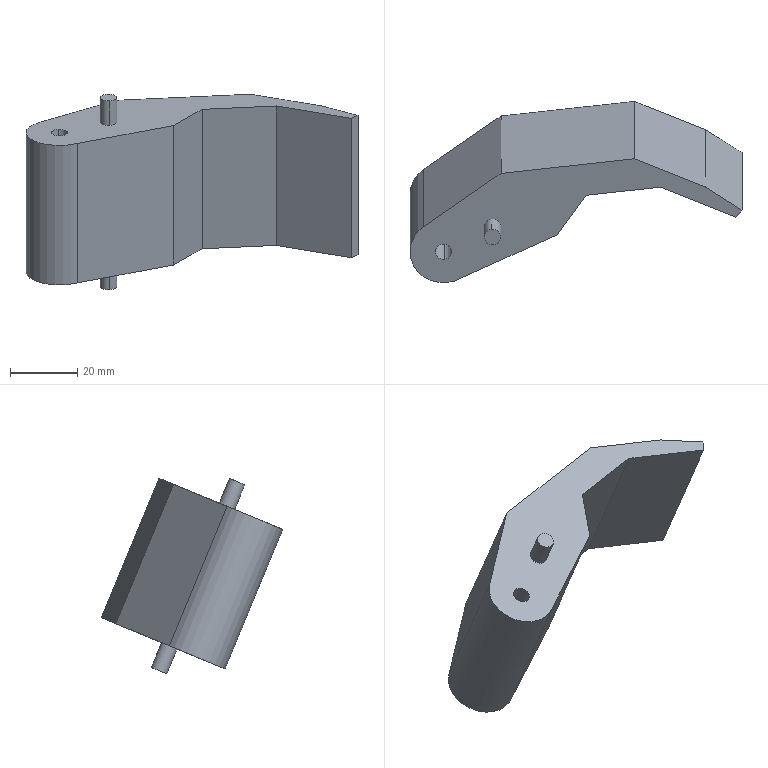Component | SolidWorks | RightJaw-1 | 1 solid | 20 faces | box 99.03 x 54.13 x 58.31 mm | volume 66368 mm3 | plane 13 | cylinder 7 | commonest cylinder face diameters 5 x6 20 x1
build123d program:
from build123d import *

# Parameters (mm, degrees)
BOSS_EXTRUDE1_DEPTH = 45
SKETCH2_R           = 2.5
CUT_EXTRUDE1_DEPTH  = 107.762
SKETCH5_R           = 2.5
BOSS_EXTRUDE3_DEPTH = 8
BOSS_EXTRUDE4_START = 8
SKETCH6_R           = 2.5
BOSS_EXTRUDE4_DEPTH = 8


with BuildPart() as part:
    # Sketch1 → Boss-Extrude1 (new body)
    with BuildSketch(Plane.XY):
        with BuildLine():
            Line((0, 0), (-14.434, -25))
            Line((-14.434, -25), (-14.434, -65))
            Line((-14.434, -65), (-2.887, -85))
            Line((-2.887, -85), (5.728, -95))
            Line((5.728, -95), (7.828, -92.858))
            Line((7.828, -92.858), (-4.434, -71.62))
            Line((-4.434, -71.62), (-4.434, -49.371))
            Line((-4.434, -49.371), (7.174, -39.371))
            Line((7.174, -39.371), (17.655, -9.371))
            ThreePointArc((17.655, -9.371), (13.349, 3.833), (0, 0))
        make_face()
    extrude(amount=BOSS_EXTRUDE1_DEPTH)

    # Sketch2 → Cut-Extrude1 (cut, through all)
    with BuildSketch(Plane.XY.offset(45)):
        with Locations((8.66, -5)):
            Circle(SKETCH2_R)
    extrude(amount=-CUT_EXTRUDE1_DEPTH, mode=Mode.SUBTRACT)

    # Sketch5 → Boss-Extrude3 (add)
    with BuildSketch(Plane.XY.offset(45)):
        with Locations(Location((2.385, -20.437, 0), (0, 0, 180))):
            Circle(SKETCH5_R)
    extrude(amount=BOSS_EXTRUDE3_DEPTH)

    # Sketch6 → Boss-Extrude4 (add)
    with BuildSketch(Plane(origin=(0, 0, 0), x_dir=(-1, 0, 0), z_dir=(0, 0, -1)).offset(BOSS_EXTRUDE4_START)):
        with Locations((-2.385, -20.437)):
            Circle(SKETCH6_R)
    extrude(amount=-BOSS_EXTRUDE4_DEPTH)


solid = part.part

# Placed as in the assembly
solid = solid.moved(Location((317.639, 27.75, 53.356), (-157.552, 0, 83.26)))
STEP:
#1=COLOUR_RGB('',0.7922,0.8196,0.9333);
#2=FILL_AREA_STYLE_COLOUR('',#1);
#3=FILL_AREA_STYLE('',(#2));
#4=SURFACE_STYLE_FILL_AREA(#3);
#5=SURFACE_SIDE_STYLE('',(#4));
#6=SURFACE_STYLE_USAGE(.BOTH.,#5);
#7=PRESENTATION_STYLE_ASSIGNMENT((#6));
#8=CARTESIAN_POINT('',(13.304,1.064,2.429));
#9=VERTEX_POINT('',#8);
#10=CARTESIAN_POINT('',(13.327,0.883,2.355));
#11=VERTEX_POINT('',#10);
#12=CARTESIAN_POINT('',(13.316,0.9733,2.392));
#13=DIRECTION('',(-0.,-0.3818,0.9242));
#14=DIRECTION('',(-0.1174,0.9178,0.3792));
#15=AXIS2_PLACEMENT_3D('',#12,#13,#14);
#16=CIRCLE('',#15,0.09843);
#17=EDGE_CURVE('',#9,#11,#16,.T.);
#18=ORIENTED_EDGE('',*,*,#17,.F.);
#19=CARTESIAN_POINT('',(13.304,1.184,2.138));
#20=VERTEX_POINT('',#19);
#21=CARTESIAN_POINT('',(13.304,1.064,2.429));
#22=DIRECTION('',(0.,0.3818,-0.9242));
#23=VECTOR('',#22,39.37);
#24=LINE('',#21,#23);
#25=EDGE_CURVE('',#9,#20,#24,.T.);
#26=ORIENTED_EDGE('',*,*,#25,.T.);
#27=CARTESIAN_POINT('',(13.327,1.003,2.064));
#28=VERTEX_POINT('',#27);
#29=CARTESIAN_POINT('',(13.316,1.094,2.101));
#30=DIRECTION('',(-0.,-0.3818,0.9242));
#31=DIRECTION('',(-0.1174,0.9178,0.3792));
#32=AXIS2_PLACEMENT_3D('',#29,#30,#31);
#33=CIRCLE('',#32,0.09843);
#34=EDGE_CURVE('',#20,#28,#33,.T.);
#35=ORIENTED_EDGE('',*,*,#34,.T.);
#36=CARTESIAN_POINT('',(13.327,0.883,2.355));
#37=DIRECTION('',(0.,0.3818,-0.9242));
#38=VECTOR('',#37,39.37);
#39=LINE('',#36,#38);
#40=EDGE_CURVE('',#11,#28,#39,.T.);
#41=ORIENTED_EDGE('',*,*,#40,.F.);
#42=EDGE_LOOP('',(#18,#26,#35,#41));
#43=FACE_OUTER_BOUND('',#42,.T.);
#44=CARTESIAN_POINT('',(13.316,0.9733,2.392));
#45=DIRECTION('',(0.,0.3818,-0.9242));
#46=DIRECTION('',(0.1174,-0.9178,-0.3792));
#47=AXIS2_PLACEMENT_3D('',#44,#45,#46);
#48=CYLINDRICAL_SURFACE('',#47,0.09843);
#49=ADVANCED_FACE('',(#43),#48,.T.);
#50=CARTESIAN_POINT('',(13.327,1.8,0.1353));
#51=VERTEX_POINT('',#50);
#52=CARTESIAN_POINT('',(13.304,1.981,0.2099));
#53=VERTEX_POINT('',#52);
#54=CARTESIAN_POINT('',(13.316,1.89,0.1726));
#55=DIRECTION('',(0.,0.3818,-0.9242));
#56=DIRECTION('',(0.1174,-0.9178,-0.3792));
#57=AXIS2_PLACEMENT_3D('',#54,#55,#56);
#58=CIRCLE('',#57,0.09843);
#59=EDGE_CURVE('',#51,#53,#58,.T.);
#60=ORIENTED_EDGE('',*,*,#59,.F.);
#61=CARTESIAN_POINT('',(13.327,1.68,0.4263));
#62=VERTEX_POINT('',#61);
#63=CARTESIAN_POINT('',(13.327,1.8,0.1353));
#64=DIRECTION('',(-0.,-0.3818,0.9242));
#65=VECTOR('',#64,39.37);
#66=LINE('',#63,#65);
#67=EDGE_CURVE('',#51,#62,#66,.T.);
#68=ORIENTED_EDGE('',*,*,#67,.T.);
#69=CARTESIAN_POINT('',(13.304,1.86,0.501));
#70=VERTEX_POINT('',#69);
#71=CARTESIAN_POINT('',(13.316,1.77,0.4637));
#72=DIRECTION('',(0.,0.3818,-0.9242));
#73=DIRECTION('',(-0.1174,0.9178,0.3792));
#74=AXIS2_PLACEMENT_3D('',#71,#72,#73);
#75=CIRCLE('',#74,0.09843);
#76=EDGE_CURVE('',#62,#70,#75,.T.);
#77=ORIENTED_EDGE('',*,*,#76,.T.);
#78=CARTESIAN_POINT('',(13.304,1.981,0.2099));
#79=DIRECTION('',(-0.,-0.3818,0.9242));
#80=VECTOR('',#79,39.37);
#81=LINE('',#78,#80);
#82=EDGE_CURVE('',#53,#70,#81,.T.);
#83=ORIENTED_EDGE('',*,*,#82,.F.);
#84=EDGE_LOOP('',(#60,#68,#77,#83));
#85=FACE_OUTER_BOUND('',#84,.T.);
#86=CARTESIAN_POINT('',(13.316,1.89,0.1726));
#87=DIRECTION('',(-0.,-0.3818,0.9242));
#88=DIRECTION('',(-0.1174,0.9178,0.3792));
#89=AXIS2_PLACEMENT_3D('',#86,#87,#88);
#90=CYLINDRICAL_SURFACE('',#89,0.09843);
#91=ADVANCED_FACE('',(#85),#90,.T.);
#92=CARTESIAN_POINT('',(12.729,0.8913,2.017));
#93=VERTEX_POINT('',#92);
#94=CARTESIAN_POINT('',(12.753,0.7106,1.943));
#95=VERTEX_POINT('',#94);
#96=CARTESIAN_POINT('',(12.741,0.8009,1.98));
#97=DIRECTION('',(0.,0.3818,-0.9242));
#98=DIRECTION('',(0.1174,-0.9178,-0.3792));
#99=AXIS2_PLACEMENT_3D('',#96,#97,#98);
#100=CIRCLE('',#99,0.09843);
#101=EDGE_CURVE('',#93,#95,#100,.T.);
#102=ORIENTED_EDGE('',*,*,#101,.F.);
#103=CARTESIAN_POINT('',(12.729,1.568,0.3801));
#104=VERTEX_POINT('',#103);
#105=CARTESIAN_POINT('',(12.729,0.8913,2.017));
#106=DIRECTION('',(0.,0.3818,-0.9242));
#107=VECTOR('',#106,39.37);
#108=LINE('',#105,#107);
#109=EDGE_CURVE('',#93,#104,#108,.T.);
#110=ORIENTED_EDGE('',*,*,#109,.T.);
#111=CARTESIAN_POINT('',(12.753,1.387,0.3054));
#112=VERTEX_POINT('',#111);
#113=CARTESIAN_POINT('',(12.741,1.477,0.3427));
#114=DIRECTION('',(0.,0.3818,-0.9242));
#115=DIRECTION('',(0.1174,-0.9178,-0.3792));
#116=AXIS2_PLACEMENT_3D('',#113,#114,#115);
#117=CIRCLE('',#116,0.09843);
#118=EDGE_CURVE('',#104,#112,#117,.T.);
#119=ORIENTED_EDGE('',*,*,#118,.T.);
#120=CARTESIAN_POINT('',(12.753,0.7106,1.943));
#121=DIRECTION('',(0.,0.3818,-0.9242));
#122=VECTOR('',#121,39.37);
#123=LINE('',#120,#122);
#124=EDGE_CURVE('',#95,#112,#123,.T.);
#125=ORIENTED_EDGE('',*,*,#124,.F.);
#126=EDGE_LOOP('',(#102,#110,#119,#125));
#127=FACE_OUTER_BOUND('',#126,.T.);
#128=CARTESIAN_POINT('',(12.741,0.8009,1.98));
#129=DIRECTION('',(0.,0.3818,-0.9242));
#130=DIRECTION('',(0.1174,-0.9178,-0.3792));
#131=AXIS2_PLACEMENT_3D('',#128,#129,#130);
#132=CYLINDRICAL_SURFACE('',#131,0.09843);
#133=ADVANCED_FACE('',(#127),#132,.F.);
#134=CARTESIAN_POINT('',(12.953,0.4946,1.854));
#135=VERTEX_POINT('',#134);
#136=CARTESIAN_POINT('',(12.505,1.093,2.101));
#137=VERTEX_POINT('',#136);
#138=CARTESIAN_POINT('',(12.741,0.8009,1.98));
#139=DIRECTION('',(0.,0.3818,-0.9242));
#140=DIRECTION('',(-0.1174,0.9178,0.3792));
#141=AXIS2_PLACEMENT_3D('',#138,#139,#140);
#142=CIRCLE('',#141,0.3937);
#143=EDGE_CURVE('',#135,#137,#142,.T.);
#144=ORIENTED_EDGE('',*,*,#143,.T.);
#145=CARTESIAN_POINT('',(12.505,1.769,0.4632));
#146=VERTEX_POINT('',#145);
#147=CARTESIAN_POINT('',(12.505,1.769,0.4632));
#148=DIRECTION('',(-0.,-0.3818,0.9242));
#149=VECTOR('',#148,39.37);
#150=LINE('',#147,#149);
#151=EDGE_CURVE('',#146,#137,#150,.T.);
#152=ORIENTED_EDGE('',*,*,#151,.F.);
#153=CARTESIAN_POINT('',(12.953,1.171,0.2162));
#154=VERTEX_POINT('',#153);
#155=CARTESIAN_POINT('',(12.741,1.477,0.3427));
#156=DIRECTION('',(0.,0.3818,-0.9242));
#157=DIRECTION('',(-0.1174,0.9178,0.3792));
#158=AXIS2_PLACEMENT_3D('',#155,#156,#157);
#159=CIRCLE('',#158,0.3937);
#160=EDGE_CURVE('',#154,#146,#159,.T.);
#161=ORIENTED_EDGE('',*,*,#160,.F.);
#162=CARTESIAN_POINT('',(12.953,1.171,0.2162));
#163=DIRECTION('',(-0.,-0.3818,0.9242));
#164=VECTOR('',#163,39.37);
#165=LINE('',#162,#164);
#166=EDGE_CURVE('',#154,#135,#165,.T.);
#167=ORIENTED_EDGE('',*,*,#166,.T.);
#168=EDGE_LOOP('',(#144,#152,#161,#167));
#169=FACE_OUTER_BOUND('',#168,.T.);
#170=CARTESIAN_POINT('',(12.741,1.477,0.3427));
#171=DIRECTION('',(-0.,-0.3818,0.9242));
#172=DIRECTION('',(-0.1174,0.9178,0.3792));
#173=AXIS2_PLACEMENT_3D('',#170,#171,#172);
#174=CYLINDRICAL_SURFACE('',#173,0.3937);
#175=ADVANCED_FACE('',(#169),#174,.T.);
#176=CARTESIAN_POINT('',(13.416,1.721,2.36));
#177=VERTEX_POINT('',#176);
#178=CARTESIAN_POINT('',(12.505,1.093,2.101));
#179=DIRECTION('',(0.8014,0.5529,0.2284));
#180=VECTOR('',#179,39.37);
#181=LINE('',#178,#180);
#182=EDGE_CURVE('',#137,#177,#181,.T.);
#183=ORIENTED_EDGE('',*,*,#182,.T.);
#184=CARTESIAN_POINT('',(13.416,2.397,0.7228));
#185=VERTEX_POINT('',#184);
#186=CARTESIAN_POINT('',(13.416,2.397,0.7228));
#187=DIRECTION('',(-0.,-0.3818,0.9242));
#188=VECTOR('',#187,39.37);
#189=LINE('',#186,#188);
#190=EDGE_CURVE('',#185,#177,#189,.T.);
#191=ORIENTED_EDGE('',*,*,#190,.F.);
#192=CARTESIAN_POINT('',(12.505,1.769,0.4632));
#193=DIRECTION('',(0.8014,0.5529,0.2284));
#194=VECTOR('',#193,39.37);
#195=LINE('',#192,#194);
#196=EDGE_CURVE('',#146,#185,#195,.T.);
#197=ORIENTED_EDGE('',*,*,#196,.F.);
#198=ORIENTED_EDGE('',*,*,#151,.T.);
#199=EDGE_LOOP('',(#183,#191,#197,#198));
#200=FACE_OUTER_BOUND('',#199,.T.);
#201=CARTESIAN_POINT('',(12.505,1.769,0.4632));
#202=DIRECTION('',(0.5982,-0.7406,-0.306));
#203=DIRECTION('',(-0.8014,-0.5529,-0.2284));
#204=AXIS2_PLACEMENT_3D('',#201,#202,#203);
#205=PLANE('',#204);
#206=ADVANCED_FACE('',(#200),#205,.F.);
#207=CARTESIAN_POINT('',(14.98,1.892,2.431));
#208=VERTEX_POINT('',#207);
#209=CARTESIAN_POINT('',(13.416,1.721,2.36));
#210=DIRECTION('',(0.9931,0.1085,0.04481));
#211=VECTOR('',#210,39.37);
#212=LINE('',#209,#211);
#213=EDGE_CURVE('',#177,#208,#212,.T.);
#214=ORIENTED_EDGE('',*,*,#213,.T.);
#215=CARTESIAN_POINT('',(14.98,2.568,0.7934));
#216=VERTEX_POINT('',#215);
#217=CARTESIAN_POINT('',(14.98,2.568,0.7934));
#218=DIRECTION('',(-0.,-0.3818,0.9242));
#219=VECTOR('',#218,39.37);
#220=LINE('',#217,#219);
#221=EDGE_CURVE('',#216,#208,#220,.T.);
#222=ORIENTED_EDGE('',*,*,#221,.F.);
#223=CARTESIAN_POINT('',(13.416,2.397,0.7228));
#224=DIRECTION('',(0.9931,0.1085,0.04481));
#225=VECTOR('',#224,39.37);
#226=LINE('',#223,#225);
#227=EDGE_CURVE('',#185,#216,#226,.T.);
#228=ORIENTED_EDGE('',*,*,#227,.F.);
#229=ORIENTED_EDGE('',*,*,#190,.T.);
#230=EDGE_LOOP('',(#214,#222,#228,#229));
#231=FACE_OUTER_BOUND('',#230,.T.);
#232=CARTESIAN_POINT('',(13.416,2.397,0.7228));
#233=DIRECTION('',(0.1174,-0.9178,-0.3792));
#234=DIRECTION('',(-0.9931,-0.1085,-0.04481));
#235=AXIS2_PLACEMENT_3D('',#232,#233,#234);
#236=PLANE('',#235);
#237=ADVANCED_FACE('',(#231),#236,.F.);
#238=CARTESIAN_POINT('',(15.815,1.56,2.294));
#239=VERTEX_POINT('',#238);
#240=CARTESIAN_POINT('',(14.98,1.892,2.431));
#241=DIRECTION('',(0.9187,-0.365,-0.1508));
#242=VECTOR('',#241,39.37);
#243=LINE('',#240,#242);
#244=EDGE_CURVE('',#208,#239,#243,.T.);
#245=ORIENTED_EDGE('',*,*,#244,.T.);
#246=CARTESIAN_POINT('',(15.815,2.236,0.6563));
#247=VERTEX_POINT('',#246);
#248=CARTESIAN_POINT('',(15.815,2.236,0.6563));
#249=DIRECTION('',(-0.,-0.3818,0.9242));
#250=VECTOR('',#249,39.37);
#251=LINE('',#248,#250);
#252=EDGE_CURVE('',#247,#239,#251,.T.);
#253=ORIENTED_EDGE('',*,*,#252,.F.);
#254=CARTESIAN_POINT('',(14.98,2.568,0.7934));
#255=DIRECTION('',(0.9187,-0.365,-0.1508));
#256=VECTOR('',#255,39.37);
#257=LINE('',#254,#256);
#258=EDGE_CURVE('',#216,#247,#257,.T.);
#259=ORIENTED_EDGE('',*,*,#258,.F.);
#260=ORIENTED_EDGE('',*,*,#221,.T.);
#261=EDGE_LOOP('',(#245,#253,#259,#260));
#262=FACE_OUTER_BOUND('',#261,.T.);
#263=CARTESIAN_POINT('',(14.98,2.568,0.7934));
#264=DIRECTION('',(-0.3949,-0.8491,-0.3508));
#265=DIRECTION('',(-0.9187,0.365,0.1508));
#266=AXIS2_PLACEMENT_3D('',#263,#264,#265);
#267=PLANE('',#266);
#268=ADVANCED_FACE('',(#262),#267,.F.);
#269=CARTESIAN_POINT('',(16.246,1.291,2.183));
#270=VERTEX_POINT('',#269);
#271=CARTESIAN_POINT('',(15.815,1.56,2.294));
#272=DIRECTION('',(0.829,-0.5169,-0.2135));
#273=VECTOR('',#272,39.37);
#274=LINE('',#271,#273);
#275=EDGE_CURVE('',#239,#270,#274,.T.);
#276=ORIENTED_EDGE('',*,*,#275,.T.);
#277=CARTESIAN_POINT('',(16.246,1.968,0.5453));
#278=VERTEX_POINT('',#277);
#279=CARTESIAN_POINT('',(16.246,1.968,0.5453));
#280=DIRECTION('',(-0.,-0.3818,0.9242));
#281=VECTOR('',#280,39.37);
#282=LINE('',#279,#281);
#283=EDGE_CURVE('',#278,#270,#282,.T.);
#284=ORIENTED_EDGE('',*,*,#283,.F.);
#285=CARTESIAN_POINT('',(15.815,2.236,0.6563));
#286=DIRECTION('',(0.829,-0.5169,-0.2135));
#287=VECTOR('',#286,39.37);
#288=LINE('',#285,#287);
#289=EDGE_CURVE('',#247,#278,#288,.T.);
#290=ORIENTED_EDGE('',*,*,#289,.F.);
#291=ORIENTED_EDGE('',*,*,#252,.T.);
#292=EDGE_LOOP('',(#276,#284,#290,#291));
#293=FACE_OUTER_BOUND('',#292,.T.);
#294=CARTESIAN_POINT('',(15.815,2.236,0.6563));
#295=DIRECTION('',(-0.5592,-0.7662,-0.3166));
#296=DIRECTION('',(-0.829,0.5169,0.2135));
#297=AXIS2_PLACEMENT_3D('',#294,#295,#296);
#298=PLANE('',#297);
#299=ADVANCED_FACE('',(#293),#298,.F.);
#300=CARTESIAN_POINT('',(16.172,1.206,2.148));
#301=VERTEX_POINT('',#300);
#302=CARTESIAN_POINT('',(16.172,1.206,2.148));
#303=DIRECTION('',(-0.627,-0.72,-0.2975));
#304=VECTOR('',#303,39.37);
#305=LINE('',#302,#304);
#306=EDGE_CURVE('',#270,#301,#305,.T.);
#307=ORIENTED_EDGE('',*,*,#306,.T.);
#308=CARTESIAN_POINT('',(16.172,1.883,0.5102));
#309=VERTEX_POINT('',#308);
#310=CARTESIAN_POINT('',(16.172,1.883,0.5102));
#311=DIRECTION('',(-0.,-0.3818,0.9242));
#312=VECTOR('',#311,39.37);
#313=LINE('',#310,#312);
#314=EDGE_CURVE('',#309,#301,#313,.T.);
#315=ORIENTED_EDGE('',*,*,#314,.F.);
#316=CARTESIAN_POINT('',(16.172,1.883,0.5102));
#317=DIRECTION('',(-0.627,-0.72,-0.2975));
#318=VECTOR('',#317,39.37);
#319=LINE('',#316,#318);
#320=EDGE_CURVE('',#278,#309,#319,.T.);
#321=ORIENTED_EDGE('',*,*,#320,.F.);
#322=ORIENTED_EDGE('',*,*,#283,.T.);
#323=EDGE_LOOP('',(#307,#315,#321,#322));
#324=FACE_OUTER_BOUND('',#323,.T.);
#325=CARTESIAN_POINT('',(16.172,1.883,0.5102));
#326=DIRECTION('',(-0.779,0.5795,0.2394));
#327=DIRECTION('',(0.627,0.72,0.2975));
#328=AXIS2_PLACEMENT_3D('',#325,#326,#327);
#329=PLANE('',#328);
#330=ADVANCED_FACE('',(#324),#329,.F.);
#331=CARTESIAN_POINT('',(15.285,1.559,2.293));
#332=VERTEX_POINT('',#331);
#333=CARTESIAN_POINT('',(15.285,1.559,2.293));
#334=DIRECTION('',(-0.9187,0.365,0.1508));
#335=VECTOR('',#334,39.37);
#336=LINE('',#333,#335);
#337=EDGE_CURVE('',#301,#332,#336,.T.);
#338=ORIENTED_EDGE('',*,*,#337,.T.);
#339=CARTESIAN_POINT('',(15.285,2.235,0.6558));
#340=VERTEX_POINT('',#339);
#341=CARTESIAN_POINT('',(15.285,2.235,0.6558));
#342=DIRECTION('',(-0.,-0.3818,0.9242));
#343=VECTOR('',#342,39.37);
#344=LINE('',#341,#343);
#345=EDGE_CURVE('',#340,#332,#344,.T.);
#346=ORIENTED_EDGE('',*,*,#345,.F.);
#347=CARTESIAN_POINT('',(15.285,2.235,0.6558));
#348=DIRECTION('',(-0.9187,0.365,0.1508));
#349=VECTOR('',#348,39.37);
#350=LINE('',#347,#349);
#351=EDGE_CURVE('',#309,#340,#350,.T.);
#352=ORIENTED_EDGE('',*,*,#351,.F.);
#353=ORIENTED_EDGE('',*,*,#314,.T.);
#354=EDGE_LOOP('',(#338,#346,#352,#353));
#355=FACE_OUTER_BOUND('',#354,.T.);
#356=CARTESIAN_POINT('',(15.285,2.235,0.6558));
#357=DIRECTION('',(0.3949,0.8491,0.3508));
#358=DIRECTION('',(0.9187,-0.365,-0.1508));
#359=AXIS2_PLACEMENT_3D('',#356,#357,#358);
#360=PLANE('',#359);
#361=ADVANCED_FACE('',(#355),#360,.F.);
#362=CARTESIAN_POINT('',(14.415,1.464,2.254));
#363=VERTEX_POINT('',#362);
#364=CARTESIAN_POINT('',(14.415,1.464,2.254));
#365=DIRECTION('',(-0.9931,-0.1085,-0.04481));
#366=VECTOR('',#365,39.37);
#367=LINE('',#364,#366);
#368=EDGE_CURVE('',#332,#363,#367,.T.);
#369=ORIENTED_EDGE('',*,*,#368,.T.);
#370=CARTESIAN_POINT('',(14.415,2.14,0.6165));
#371=VERTEX_POINT('',#370);
#372=CARTESIAN_POINT('',(14.415,2.14,0.6165));
#373=DIRECTION('',(-0.,-0.3818,0.9242));
#374=VECTOR('',#373,39.37);
#375=LINE('',#372,#374);
#376=EDGE_CURVE('',#371,#363,#375,.T.);
#377=ORIENTED_EDGE('',*,*,#376,.F.);
#378=CARTESIAN_POINT('',(14.415,2.14,0.6165));
#379=DIRECTION('',(-0.9931,-0.1085,-0.04481));
#380=VECTOR('',#379,39.37);
#381=LINE('',#378,#380);
#382=EDGE_CURVE('',#340,#371,#381,.T.);
#383=ORIENTED_EDGE('',*,*,#382,.F.);
#384=ORIENTED_EDGE('',*,*,#345,.T.);
#385=EDGE_LOOP('',(#369,#377,#383,#384));
#386=FACE_OUTER_BOUND('',#385,.T.);
#387=CARTESIAN_POINT('',(14.415,2.14,0.6165));
#388=DIRECTION('',(-0.1174,0.9178,0.3792));
#389=DIRECTION('',(0.9931,0.1085,0.04481));
#390=AXIS2_PLACEMENT_3D('',#387,#388,#389);
#391=PLANE('',#390);
#392=ADVANCED_FACE('',(#386),#391,.F.);
#393=CARTESIAN_POINT('',(14.078,1.001,2.063));
#394=VERTEX_POINT('',#393);
#395=CARTESIAN_POINT('',(14.078,1.001,2.063));
#396=DIRECTION('',(-0.5592,-0.7662,-0.3166));
#397=VECTOR('',#396,39.37);
#398=LINE('',#395,#397);
#399=EDGE_CURVE('',#363,#394,#398,.T.);
#400=ORIENTED_EDGE('',*,*,#399,.T.);
#401=CARTESIAN_POINT('',(14.078,1.678,0.4256));
#402=VERTEX_POINT('',#401);
#403=CARTESIAN_POINT('',(14.078,1.678,0.4256));
#404=DIRECTION('',(-0.,-0.3818,0.9242));
#405=VECTOR('',#404,39.37);
#406=LINE('',#403,#405);
#407=EDGE_CURVE('',#402,#394,#406,.T.);
#408=ORIENTED_EDGE('',*,*,#407,.F.);
#409=CARTESIAN_POINT('',(14.078,1.678,0.4256));
#410=DIRECTION('',(-0.5592,-0.7662,-0.3166));
#411=VECTOR('',#410,39.37);
#412=LINE('',#409,#411);
#413=EDGE_CURVE('',#371,#402,#412,.T.);
#414=ORIENTED_EDGE('',*,*,#413,.F.);
#415=ORIENTED_EDGE('',*,*,#376,.T.);
#416=EDGE_LOOP('',(#400,#408,#414,#415));
#417=FACE_OUTER_BOUND('',#416,.T.);
#418=CARTESIAN_POINT('',(14.078,1.678,0.4256));
#419=DIRECTION('',(-0.829,0.5169,0.2135));
#420=DIRECTION('',(0.5592,0.7662,0.3166));
#421=AXIS2_PLACEMENT_3D('',#418,#419,#420);
#422=PLANE('',#421);
#423=ADVANCED_FACE('',(#417),#422,.F.);
#424=CARTESIAN_POINT('',(12.953,0.4946,1.854));
#425=DIRECTION('',(-0.8988,-0.4051,-0.1674));
#426=VECTOR('',#425,39.37);
#427=LINE('',#424,#426);
#428=EDGE_CURVE('',#394,#135,#427,.T.);
#429=ORIENTED_EDGE('',*,*,#428,.T.);
#430=ORIENTED_EDGE('',*,*,#166,.F.);
#431=CARTESIAN_POINT('',(12.953,1.171,0.2162));
#432=DIRECTION('',(-0.8988,-0.4051,-0.1674));
#433=VECTOR('',#432,39.37);
#434=LINE('',#431,#433);
#435=EDGE_CURVE('',#402,#154,#434,.T.);
#436=ORIENTED_EDGE('',*,*,#435,.F.);
#437=ORIENTED_EDGE('',*,*,#407,.T.);
#438=EDGE_LOOP('',(#429,#430,#436,#437));
#439=FACE_OUTER_BOUND('',#438,.T.);
#440=CARTESIAN_POINT('',(12.953,1.171,0.2162));
#441=DIRECTION('',(-0.4383,0.8307,0.3432));
#442=DIRECTION('',(0.8988,0.4051,0.1674));
#443=AXIS2_PLACEMENT_3D('',#440,#441,#442);
#444=PLANE('',#443);
#445=ADVANCED_FACE('',(#439),#444,.F.);
#446=CARTESIAN_POINT('',(13.316,1.77,0.4637));
#447=DIRECTION('',(0.,0.3818,-0.9242));
#448=DIRECTION('',(-0.1174,0.9178,0.3792));
#449=AXIS2_PLACEMENT_3D('',#446,#447,#448);
#450=CIRCLE('',#449,0.09843);
#451=EDGE_CURVE('',#70,#62,#450,.T.);
#452=ORIENTED_EDGE('',*,*,#451,.F.);
#453=ORIENTED_EDGE('',*,*,#76,.F.);
#454=EDGE_LOOP('',(#452,#453));
#455=FACE_BOUND('',#454,.T.);
#456=CARTESIAN_POINT('',(12.741,1.477,0.3427));
#457=DIRECTION('',(0.,0.3818,-0.9242));
#458=DIRECTION('',(0.1174,-0.9178,-0.3792));
#459=AXIS2_PLACEMENT_3D('',#456,#457,#458);
#460=CIRCLE('',#459,0.09843);
#461=EDGE_CURVE('',#112,#104,#460,.T.);
#462=ORIENTED_EDGE('',*,*,#461,.F.);
#463=ORIENTED_EDGE('',*,*,#118,.F.);
#464=EDGE_LOOP('',(#462,#463));
#465=FACE_BOUND('',#464,.T.);
#466=ORIENTED_EDGE('',*,*,#160,.T.);
#467=ORIENTED_EDGE('',*,*,#196,.T.);
#468=ORIENTED_EDGE('',*,*,#227,.T.);
#469=ORIENTED_EDGE('',*,*,#258,.T.);
#470=ORIENTED_EDGE('',*,*,#289,.T.);
#471=ORIENTED_EDGE('',*,*,#320,.T.);
#472=ORIENTED_EDGE('',*,*,#351,.T.);
#473=ORIENTED_EDGE('',*,*,#382,.T.);
#474=ORIENTED_EDGE('',*,*,#413,.T.);
#475=ORIENTED_EDGE('',*,*,#435,.T.);
#476=EDGE_LOOP('',(#466,#467,#468,#469,#470,#471,#472,#473,#474,#475));
#477=FACE_OUTER_BOUND('',#476,.T.);
#478=CARTESIAN_POINT('',(12.741,1.477,0.3427));
#479=DIRECTION('',(-0.,-0.3818,0.9242));
#480=DIRECTION('',(-0.1174,0.9178,0.3792));
#481=AXIS2_PLACEMENT_3D('',#478,#479,#480);
#482=PLANE('',#481);
#483=ADVANCED_FACE('',(#455,#465,#477),#482,.F.);
#484=CARTESIAN_POINT('',(13.316,1.094,2.101));
#485=DIRECTION('',(-0.,-0.3818,0.9242));
#486=DIRECTION('',(-0.1174,0.9178,0.3792));
#487=AXIS2_PLACEMENT_3D('',#484,#485,#486);
#488=CIRCLE('',#487,0.09843);
#489=EDGE_CURVE('',#28,#20,#488,.T.);
#490=ORIENTED_EDGE('',*,*,#489,.F.);
#491=ORIENTED_EDGE('',*,*,#34,.F.);
#492=EDGE_LOOP('',(#490,#491));
#493=FACE_BOUND('',#492,.T.);
#494=CARTESIAN_POINT('',(12.741,0.8009,1.98));
#495=DIRECTION('',(0.,0.3818,-0.9242));
#496=DIRECTION('',(0.1174,-0.9178,-0.3792));
#497=AXIS2_PLACEMENT_3D('',#494,#495,#496);
#498=CIRCLE('',#497,0.09843);
#499=EDGE_CURVE('',#95,#93,#498,.T.);
#500=ORIENTED_EDGE('',*,*,#499,.T.);
#501=ORIENTED_EDGE('',*,*,#101,.T.);
#502=EDGE_LOOP('',(#500,#501));
#503=FACE_BOUND('',#502,.T.);
#504=ORIENTED_EDGE('',*,*,#143,.F.);
#505=ORIENTED_EDGE('',*,*,#428,.F.);
#506=ORIENTED_EDGE('',*,*,#399,.F.);
#507=ORIENTED_EDGE('',*,*,#368,.F.);
#508=ORIENTED_EDGE('',*,*,#337,.F.);
#509=ORIENTED_EDGE('',*,*,#306,.F.);
#510=ORIENTED_EDGE('',*,*,#275,.F.);
#511=ORIENTED_EDGE('',*,*,#244,.F.);
#512=ORIENTED_EDGE('',*,*,#213,.F.);
#513=ORIENTED_EDGE('',*,*,#182,.F.);
#514=EDGE_LOOP('',(#504,#505,#506,#507,#508,#509,#510,#511,#512,#513));
#515=FACE_OUTER_BOUND('',#514,.T.);
#516=CARTESIAN_POINT('',(12.741,0.8009,1.98));
#517=DIRECTION('',(-0.,-0.3818,0.9242));
#518=DIRECTION('',(-0.1174,0.9178,0.3792));
#519=AXIS2_PLACEMENT_3D('',#516,#517,#518);
#520=PLANE('',#519);
#521=ADVANCED_FACE('',(#493,#503,#515),#520,.T.);
#522=ORIENTED_EDGE('',*,*,#109,.F.);
#523=ORIENTED_EDGE('',*,*,#499,.F.);
#524=ORIENTED_EDGE('',*,*,#124,.T.);
#525=ORIENTED_EDGE('',*,*,#461,.T.);
#526=EDGE_LOOP('',(#522,#523,#524,#525));
#527=FACE_OUTER_BOUND('',#526,.T.);
#528=CARTESIAN_POINT('',(12.741,0.8009,1.98));
#529=DIRECTION('',(0.,0.3818,-0.9242));
#530=DIRECTION('',(0.1174,-0.9178,-0.3792));
#531=AXIS2_PLACEMENT_3D('',#528,#529,#530);
#532=CYLINDRICAL_SURFACE('',#531,0.09843);
#533=ADVANCED_FACE('',(#527),#532,.F.);
#534=ORIENTED_EDGE('',*,*,#67,.F.);
#535=CARTESIAN_POINT('',(13.316,1.89,0.1726));
#536=DIRECTION('',(0.,0.3818,-0.9242));
#537=DIRECTION('',(0.1174,-0.9178,-0.3792));
#538=AXIS2_PLACEMENT_3D('',#535,#536,#537);
#539=CIRCLE('',#538,0.09843);
#540=EDGE_CURVE('',#53,#51,#539,.T.);
#541=ORIENTED_EDGE('',*,*,#540,.F.);
#542=ORIENTED_EDGE('',*,*,#82,.T.);
#543=ORIENTED_EDGE('',*,*,#451,.T.);
#544=EDGE_LOOP('',(#534,#541,#542,#543));
#545=FACE_OUTER_BOUND('',#544,.T.);
#546=CARTESIAN_POINT('',(13.316,1.89,0.1726));
#547=DIRECTION('',(-0.,-0.3818,0.9242));
#548=DIRECTION('',(-0.1174,0.9178,0.3792));
#549=AXIS2_PLACEMENT_3D('',#546,#547,#548);
#550=CYLINDRICAL_SURFACE('',#549,0.09843);
#551=ADVANCED_FACE('',(#545),#550,.T.);
#552=ORIENTED_EDGE('',*,*,#540,.T.);
#553=ORIENTED_EDGE('',*,*,#59,.T.);
#554=EDGE_LOOP('',(#552,#553));
#555=FACE_OUTER_BOUND('',#554,.T.);
#556=CARTESIAN_POINT('',(13.316,1.89,0.1726));
#557=DIRECTION('',(0.,0.3818,-0.9242));
#558=DIRECTION('',(0.1174,-0.9178,-0.3792));
#559=AXIS2_PLACEMENT_3D('',#556,#557,#558);
#560=PLANE('',#559);
#561=ADVANCED_FACE('',(#555),#560,.T.);
#562=ORIENTED_EDGE('',*,*,#25,.F.);
#563=CARTESIAN_POINT('',(13.316,0.9733,2.392));
#564=DIRECTION('',(-0.,-0.3818,0.9242));
#565=DIRECTION('',(-0.1174,0.9178,0.3792));
#566=AXIS2_PLACEMENT_3D('',#563,#564,#565);
#567=CIRCLE('',#566,0.09843);
#568=EDGE_CURVE('',#11,#9,#567,.T.);
#569=ORIENTED_EDGE('',*,*,#568,.F.);
#570=ORIENTED_EDGE('',*,*,#40,.T.);
#571=ORIENTED_EDGE('',*,*,#489,.T.);
#572=EDGE_LOOP('',(#562,#569,#570,#571));
#573=FACE_OUTER_BOUND('',#572,.T.);
#574=CARTESIAN_POINT('',(13.316,0.9733,2.392));
#575=DIRECTION('',(0.,0.3818,-0.9242));
#576=DIRECTION('',(0.1174,-0.9178,-0.3792));
#577=AXIS2_PLACEMENT_3D('',#574,#575,#576);
#578=CYLINDRICAL_SURFACE('',#577,0.09843);
#579=ADVANCED_FACE('',(#573),#578,.T.);
#580=ORIENTED_EDGE('',*,*,#568,.T.);
#581=ORIENTED_EDGE('',*,*,#17,.T.);
#582=EDGE_LOOP('',(#580,#581));
#583=FACE_OUTER_BOUND('',#582,.T.);
#584=CARTESIAN_POINT('',(13.316,0.9733,2.392));
#585=DIRECTION('',(-0.,-0.3818,0.9242));
#586=DIRECTION('',(-0.1174,0.9178,0.3792));
#587=AXIS2_PLACEMENT_3D('',#584,#585,#586);
#588=PLANE('',#587);
#589=ADVANCED_FACE('',(#583),#588,.T.);
#590=CLOSED_SHELL('',(#49,#91,#133,#175,#206,#237,#268,#299,#330,#361,#392,#423,#445,#483,#521,#533,#551,#561,#579,#589));
#591=MANIFOLD_SOLID_BREP('',#590);
#592=STYLED_ITEM('',(#7),#591);
#593=(LENGTH_UNIT()NAMED_UNIT(*)SI_UNIT($,.METRE.));
#594=LENGTH_MEASURE_WITH_UNIT(LENGTH_MEASURE(0.0254),#593);
#595=DIMENSIONAL_EXPONENTS(1.,0.,0.,0.,0.,0.,0.);
#596=(CONVERSION_BASED_UNIT('',#594)LENGTH_UNIT()NAMED_UNIT(#595));
#597=UNCERTAINTY_MEASURE_WITH_UNIT(LENGTH_MEASURE(0.00001),#596,'','');
#598=(NAMED_UNIT(*)PLANE_ANGLE_UNIT()SI_UNIT($,.RADIAN.));
#599=(NAMED_UNIT(*)SI_UNIT($,.STERADIAN.)SOLID_ANGLE_UNIT());
#600=(GEOMETRIC_REPRESENTATION_CONTEXT(3)GLOBAL_UNCERTAINTY_ASSIGNED_CONTEXT((#597))GLOBAL_UNIT_ASSIGNED_CONTEXT((#596,#598,#599))REPRESENTATION_CONTEXT('',''));
#601=MECHANICAL_DESIGN_GEOMETRIC_PRESENTATION_REPRESENTATION('',(#592),#600);
#602=PRESENTATION_LAYER_ASSIGNMENT('','',(#592));
#603=CARTESIAN_POINT('',(0.,0.,0.));
#604=DIRECTION('',(0.,0.,1.));
#605=DIRECTION('',(1.,0.,0.));
#606=AXIS2_PLACEMENT_3D('',#603,#604,#605);
#607=(LENGTH_UNIT()NAMED_UNIT(*)SI_UNIT($,.METRE.));
#608=LENGTH_MEASURE_WITH_UNIT(LENGTH_MEASURE(0.0254),#607);
#609=DIMENSIONAL_EXPONENTS(1.,0.,0.,0.,0.,0.,0.);
#610=(CONVERSION_BASED_UNIT('',#608)LENGTH_UNIT()NAMED_UNIT(#609));
#611=UNCERTAINTY_MEASURE_WITH_UNIT(LENGTH_MEASURE(0.00001),#610,'','');
#612=(NAMED_UNIT(*)PLANE_ANGLE_UNIT()SI_UNIT($,.RADIAN.));
#613=(NAMED_UNIT(*)SI_UNIT($,.STERADIAN.)SOLID_ANGLE_UNIT());
#614=(GEOMETRIC_REPRESENTATION_CONTEXT(3)GLOBAL_UNCERTAINTY_ASSIGNED_CONTEXT((#611))GLOBAL_UNIT_ASSIGNED_CONTEXT((#610,#612,#613))REPRESENTATION_CONTEXT('',''));
#615=ADVANCED_BREP_SHAPE_REPRESENTATION('',(#591,#606),#614);